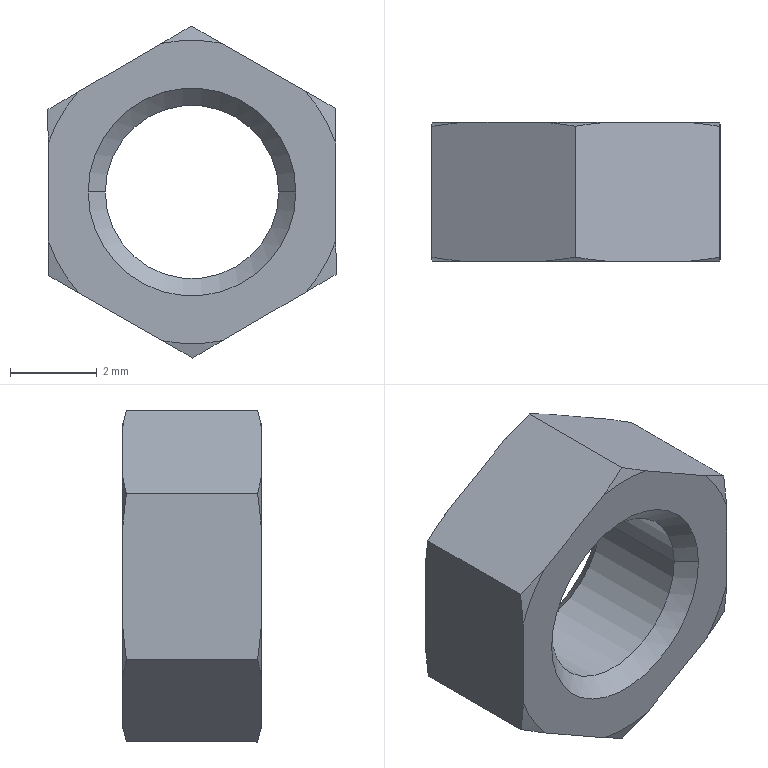Component | SolidWorks | GB_T6170-2000Type1HexNutGradeAAndBM4-1 | 1 solid | 26 faces | box 6.65 x 3.2 x 7.66 mm | volume 80 mm3 | cone 16 | plane 8 | cylinder 2 | commonest cylinder face diameters 4 x2
STEP:
#1=COLOUR_RGB('',0.7922,0.8196,0.9333);
#2=FILL_AREA_STYLE_COLOUR('',#1);
#3=FILL_AREA_STYLE('',(#2));
#4=SURFACE_STYLE_FILL_AREA(#3);
#5=SURFACE_SIDE_STYLE('',(#4));
#6=SURFACE_STYLE_USAGE(.BOTH.,#5);
#7=PRESENTATION_STYLE_ASSIGNMENT((#6));
#8=CARTESIAN_POINT('',(-5.651,2.991,-5.768));
#9=VERTEX_POINT('',#8);
#10=CARTESIAN_POINT('',(-5.493,2.991,-5.768));
#11=VERTEX_POINT('',#10);
#12=CARTESIAN_POINT('',(-5.572,2.991,-5.768));
#13=DIRECTION('',(0.,1.,0.));
#14=DIRECTION('',(-1.,0.,0.));
#15=AXIS2_PLACEMENT_3D('',#12,#13,#14);
#16=CIRCLE('',#15,0.07874);
#17=EDGE_CURVE('',#9,#11,#16,.T.);
#18=ORIENTED_EDGE('',*,*,#17,.F.);
#19=CARTESIAN_POINT('',(-5.667,3.007,-5.768));
#20=VERTEX_POINT('',#19);
#21=CARTESIAN_POINT('',(-5.651,2.991,-5.768));
#22=DIRECTION('',(-0.7071,0.7071,-0.));
#23=VECTOR('',#22,39.37);
#24=LINE('',#21,#23);
#25=EDGE_CURVE('',#9,#20,#24,.T.);
#26=ORIENTED_EDGE('',*,*,#25,.T.);
#27=CARTESIAN_POINT('',(-5.478,3.007,-5.768));
#28=VERTEX_POINT('',#27);
#29=CARTESIAN_POINT('',(-5.572,3.007,-5.768));
#30=DIRECTION('',(0.,-1.,0.));
#31=DIRECTION('',(-1.,0.,0.));
#32=AXIS2_PLACEMENT_3D('',#29,#30,#31);
#33=CIRCLE('',#32,0.0943);
#34=EDGE_CURVE('',#28,#20,#33,.T.);
#35=ORIENTED_EDGE('',*,*,#34,.F.);
#36=CARTESIAN_POINT('',(-5.493,2.991,-5.768));
#37=DIRECTION('',(0.7071,0.7071,0.));
#38=VECTOR('',#37,39.37);
#39=LINE('',#36,#38);
#40=EDGE_CURVE('',#11,#28,#39,.T.);
#41=ORIENTED_EDGE('',*,*,#40,.F.);
#42=EDGE_LOOP('',(#18,#26,#35,#41));
#43=FACE_OUTER_BOUND('',#42,.T.);
#44=CARTESIAN_POINT('',(-5.572,2.991,-5.768));
#45=DIRECTION('',(0.,1.,0.));
#46=DIRECTION('',(1.,0.,0.));
#47=AXIS2_PLACEMENT_3D('',#44,#45,#46);
#48=CONICAL_SURFACE('',#47,0.07874,0.7854);
#49=ADVANCED_FACE('',(#43),#48,.F.);
#50=CARTESIAN_POINT('',(-5.493,2.896,-5.768));
#51=VERTEX_POINT('',#50);
#52=CARTESIAN_POINT('',(-5.651,2.896,-5.768));
#53=VERTEX_POINT('',#52);
#54=CARTESIAN_POINT('',(-5.572,2.896,-5.768));
#55=DIRECTION('',(0.,-1.,0.));
#56=DIRECTION('',(-1.,0.,0.));
#57=AXIS2_PLACEMENT_3D('',#54,#55,#56);
#58=CIRCLE('',#57,0.07874);
#59=EDGE_CURVE('',#51,#53,#58,.T.);
#60=ORIENTED_EDGE('',*,*,#59,.F.);
#61=CARTESIAN_POINT('',(-5.478,2.881,-5.768));
#62=VERTEX_POINT('',#61);
#63=CARTESIAN_POINT('',(-5.478,2.881,-5.768));
#64=DIRECTION('',(0.7071,-0.7071,-0.));
#65=VECTOR('',#64,39.37);
#66=LINE('',#63,#65);
#67=EDGE_CURVE('',#51,#62,#66,.T.);
#68=ORIENTED_EDGE('',*,*,#67,.T.);
#69=CARTESIAN_POINT('',(-5.667,2.881,-5.768));
#70=VERTEX_POINT('',#69);
#71=CARTESIAN_POINT('',(-5.572,2.881,-5.768));
#72=DIRECTION('',(0.,1.,0.));
#73=DIRECTION('',(-1.,0.,0.));
#74=AXIS2_PLACEMENT_3D('',#71,#72,#73);
#75=CIRCLE('',#74,0.0943);
#76=EDGE_CURVE('',#70,#62,#75,.T.);
#77=ORIENTED_EDGE('',*,*,#76,.F.);
#78=CARTESIAN_POINT('',(-5.667,2.881,-5.768));
#79=DIRECTION('',(-0.7071,-0.7071,0.));
#80=VECTOR('',#79,39.37);
#81=LINE('',#78,#80);
#82=EDGE_CURVE('',#53,#70,#81,.T.);
#83=ORIENTED_EDGE('',*,*,#82,.F.);
#84=EDGE_LOOP('',(#60,#68,#77,#83));
#85=FACE_OUTER_BOUND('',#84,.T.);
#86=CARTESIAN_POINT('',(-5.572,2.881,-5.768));
#87=DIRECTION('',(0.,-1.,0.));
#88=DIRECTION('',(-1.,0.,0.));
#89=AXIS2_PLACEMENT_3D('',#86,#87,#88);
#90=CONICAL_SURFACE('',#89,0.0943,0.7854);
#91=ADVANCED_FACE('',(#85),#90,.F.);
#92=ORIENTED_EDGE('',*,*,#17,.T.);
#93=CARTESIAN_POINT('',(-5.493,3.007,-5.768));
#94=DIRECTION('',(0.,-1.,0.));
#95=VECTOR('',#94,39.37);
#96=LINE('',#93,#95);
#97=EDGE_CURVE('',#11,#51,#96,.T.);
#98=ORIENTED_EDGE('',*,*,#97,.T.);
#99=ORIENTED_EDGE('',*,*,#59,.T.);
#100=CARTESIAN_POINT('',(-5.651,3.007,-5.768));
#101=DIRECTION('',(0.,-1.,0.));
#102=VECTOR('',#101,39.37);
#103=LINE('',#100,#102);
#104=EDGE_CURVE('',#9,#53,#103,.T.);
#105=ORIENTED_EDGE('',*,*,#104,.F.);
#106=EDGE_LOOP('',(#92,#98,#99,#105));
#107=FACE_OUTER_BOUND('',#106,.T.);
#108=CARTESIAN_POINT('',(-5.572,3.007,-5.768));
#109=DIRECTION('',(0.,-1.,0.));
#110=DIRECTION('',(-1.,0.,0.));
#111=AXIS2_PLACEMENT_3D('',#108,#109,#110);
#112=CYLINDRICAL_SURFACE('',#111,0.07874);
#113=ADVANCED_FACE('',(#107),#112,.F.);
#114=CARTESIAN_POINT('',(-5.441,3.003,-5.843));
#115=VERTEX_POINT('',#114);
#116=CARTESIAN_POINT('',(-5.468,3.007,-5.859));
#117=VERTEX_POINT('',#116);
#118=CARTESIAN_POINT('',(-5.441,3.003,-5.843));
#119=CARTESIAN_POINT('',(-5.45,3.004,-5.848));
#120=CARTESIAN_POINT('',(-5.459,3.006,-5.853));
#121=CARTESIAN_POINT('',(-5.468,3.007,-5.859));
#122=B_SPLINE_CURVE_WITH_KNOTS('',3,(#118,#119,#120,#121),.UNSPECIFIED.,.F.,.F.,(4,4),(0.00352,0.004323),.UNSPECIFIED.);
#123=EDGE_CURVE('',#115,#117,#122,.T.);
#124=ORIENTED_EDGE('',*,*,#123,.F.);
#125=CARTESIAN_POINT('',(-5.441,2.884,-5.843));
#126=VERTEX_POINT('',#125);
#127=CARTESIAN_POINT('',(-5.441,3.007,-5.843));
#128=DIRECTION('',(0.,-1.,0.));
#129=VECTOR('',#128,39.37);
#130=LINE('',#127,#129);
#131=EDGE_CURVE('',#115,#126,#130,.T.);
#132=ORIENTED_EDGE('',*,*,#131,.T.);
#133=CARTESIAN_POINT('',(-5.468,2.881,-5.859));
#134=VERTEX_POINT('',#133);
#135=CARTESIAN_POINT('',(-5.468,2.881,-5.859));
#136=CARTESIAN_POINT('',(-5.459,2.881,-5.853));
#137=CARTESIAN_POINT('',(-5.45,2.883,-5.848));
#138=CARTESIAN_POINT('',(-5.441,2.884,-5.843));
#139=B_SPLINE_CURVE_WITH_KNOTS('',3,(#135,#136,#137,#138),.UNSPECIFIED.,.F.,.F.,(4,4),(0.006542,0.007331),.UNSPECIFIED.);
#140=EDGE_CURVE('',#134,#126,#139,.T.);
#141=ORIENTED_EDGE('',*,*,#140,.F.);
#142=CARTESIAN_POINT('',(-5.544,2.881,-5.903));
#143=VERTEX_POINT('',#142);
#144=CARTESIAN_POINT('',(-5.441,2.881,-5.843));
#145=DIRECTION('',(-0.8641,0.,-0.5034));
#146=VECTOR('',#145,39.37);
#147=LINE('',#144,#146);
#148=EDGE_CURVE('',#134,#143,#147,.T.);
#149=ORIENTED_EDGE('',*,*,#148,.T.);
#150=CARTESIAN_POINT('',(-5.572,2.884,-5.919));
#151=VERTEX_POINT('',#150);
#152=CARTESIAN_POINT('',(-5.572,2.884,-5.919));
#153=CARTESIAN_POINT('',(-5.563,2.883,-5.914));
#154=CARTESIAN_POINT('',(-5.554,2.881,-5.908));
#155=CARTESIAN_POINT('',(-5.544,2.881,-5.903));
#156=B_SPLINE_CURVE_WITH_KNOTS('',3,(#152,#153,#154,#155),.UNSPECIFIED.,.F.,.F.,(4,4),(0.00352,0.004323),.UNSPECIFIED.);
#157=EDGE_CURVE('',#151,#143,#156,.T.);
#158=ORIENTED_EDGE('',*,*,#157,.F.);
#159=CARTESIAN_POINT('',(-5.572,3.003,-5.919));
#160=VERTEX_POINT('',#159);
#161=CARTESIAN_POINT('',(-5.572,3.007,-5.919));
#162=DIRECTION('',(0.,-1.,0.));
#163=VECTOR('',#162,39.37);
#164=LINE('',#161,#163);
#165=EDGE_CURVE('',#160,#151,#164,.T.);
#166=ORIENTED_EDGE('',*,*,#165,.F.);
#167=CARTESIAN_POINT('',(-5.544,3.007,-5.903));
#168=VERTEX_POINT('',#167);
#169=CARTESIAN_POINT('',(-5.544,3.007,-5.903));
#170=CARTESIAN_POINT('',(-5.554,3.006,-5.908));
#171=CARTESIAN_POINT('',(-5.563,3.004,-5.914));
#172=CARTESIAN_POINT('',(-5.572,3.003,-5.919));
#173=B_SPLINE_CURVE_WITH_KNOTS('',3,(#169,#170,#171,#172),.UNSPECIFIED.,.F.,.F.,(4,4),(0.006542,0.007331),.UNSPECIFIED.);
#174=EDGE_CURVE('',#168,#160,#173,.T.);
#175=ORIENTED_EDGE('',*,*,#174,.F.);
#176=CARTESIAN_POINT('',(-5.441,3.007,-5.843));
#177=DIRECTION('',(-0.8641,0.,-0.5034));
#178=VECTOR('',#177,39.37);
#179=LINE('',#176,#178);
#180=EDGE_CURVE('',#117,#168,#179,.T.);
#181=ORIENTED_EDGE('',*,*,#180,.F.);
#182=EDGE_LOOP('',(#124,#132,#141,#149,#158,#166,#175,#181));
#183=FACE_OUTER_BOUND('',#182,.T.);
#184=CARTESIAN_POINT('',(-5.441,3.007,-5.843));
#185=DIRECTION('',(-0.5034,0.,0.8641));
#186=DIRECTION('',(0.8641,0.,0.5034));
#187=AXIS2_PLACEMENT_3D('',#184,#185,#186);
#188=PLANE('',#187);
#189=ADVANCED_FACE('',(#183),#188,.F.);
#190=CARTESIAN_POINT('',(-5.599,3.007,-5.903));
#191=VERTEX_POINT('',#190);
#192=CARTESIAN_POINT('',(-5.572,3.003,-5.919));
#193=CARTESIAN_POINT('',(-5.581,3.004,-5.914));
#194=CARTESIAN_POINT('',(-5.59,3.006,-5.908));
#195=CARTESIAN_POINT('',(-5.599,3.007,-5.903));
#196=B_SPLINE_CURVE_WITH_KNOTS('',3,(#192,#193,#194,#195),.UNSPECIFIED.,.F.,.F.,(4,4),(0.003504,0.004307),.UNSPECIFIED.);
#197=EDGE_CURVE('',#160,#191,#196,.T.);
#198=ORIENTED_EDGE('',*,*,#197,.F.);
#199=ORIENTED_EDGE('',*,*,#165,.T.);
#200=CARTESIAN_POINT('',(-5.599,2.881,-5.903));
#201=VERTEX_POINT('',#200);
#202=CARTESIAN_POINT('',(-5.599,2.881,-5.903));
#203=CARTESIAN_POINT('',(-5.59,2.881,-5.908));
#204=CARTESIAN_POINT('',(-5.581,2.883,-5.914));
#205=CARTESIAN_POINT('',(-5.572,2.884,-5.919));
#206=B_SPLINE_CURVE_WITH_KNOTS('',3,(#202,#203,#204,#205),.UNSPECIFIED.,.F.,.F.,(4,4),(0.006526,0.007315),.UNSPECIFIED.);
#207=EDGE_CURVE('',#201,#151,#206,.T.);
#208=ORIENTED_EDGE('',*,*,#207,.F.);
#209=CARTESIAN_POINT('',(-5.675,2.881,-5.859));
#210=VERTEX_POINT('',#209);
#211=CARTESIAN_POINT('',(-5.572,2.881,-5.919));
#212=DIRECTION('',(-0.868,0.,0.4966));
#213=VECTOR('',#212,39.37);
#214=LINE('',#211,#213);
#215=EDGE_CURVE('',#201,#210,#214,.T.);
#216=ORIENTED_EDGE('',*,*,#215,.T.);
#217=CARTESIAN_POINT('',(-5.703,2.884,-5.844));
#218=VERTEX_POINT('',#217);
#219=CARTESIAN_POINT('',(-5.703,2.884,-5.844));
#220=CARTESIAN_POINT('',(-5.693,2.883,-5.849));
#221=CARTESIAN_POINT('',(-5.684,2.881,-5.854));
#222=CARTESIAN_POINT('',(-5.675,2.881,-5.859));
#223=B_SPLINE_CURVE_WITH_KNOTS('',3,(#219,#220,#221,#222),.UNSPECIFIED.,.F.,.F.,(4,4),(0.003504,0.004307),.UNSPECIFIED.);
#224=EDGE_CURVE('',#218,#210,#223,.T.);
#225=ORIENTED_EDGE('',*,*,#224,.F.);
#226=CARTESIAN_POINT('',(-5.703,3.003,-5.844));
#227=VERTEX_POINT('',#226);
#228=CARTESIAN_POINT('',(-5.703,3.007,-5.844));
#229=DIRECTION('',(0.,-1.,0.));
#230=VECTOR('',#229,39.37);
#231=LINE('',#228,#230);
#232=EDGE_CURVE('',#227,#218,#231,.T.);
#233=ORIENTED_EDGE('',*,*,#232,.F.);
#234=CARTESIAN_POINT('',(-5.675,3.007,-5.859));
#235=VERTEX_POINT('',#234);
#236=CARTESIAN_POINT('',(-5.675,3.007,-5.859));
#237=CARTESIAN_POINT('',(-5.684,3.006,-5.854));
#238=CARTESIAN_POINT('',(-5.693,3.004,-5.849));
#239=CARTESIAN_POINT('',(-5.703,3.003,-5.844));
#240=B_SPLINE_CURVE_WITH_KNOTS('',3,(#236,#237,#238,#239),.UNSPECIFIED.,.F.,.F.,(4,4),(0.006526,0.007315),.UNSPECIFIED.);
#241=EDGE_CURVE('',#235,#227,#240,.T.);
#242=ORIENTED_EDGE('',*,*,#241,.F.);
#243=CARTESIAN_POINT('',(-5.572,3.007,-5.919));
#244=DIRECTION('',(-0.868,0.,0.4966));
#245=VECTOR('',#244,39.37);
#246=LINE('',#243,#245);
#247=EDGE_CURVE('',#191,#235,#246,.T.);
#248=ORIENTED_EDGE('',*,*,#247,.F.);
#249=EDGE_LOOP('',(#198,#199,#208,#216,#225,#233,#242,#248));
#250=FACE_OUTER_BOUND('',#249,.T.);
#251=CARTESIAN_POINT('',(-5.572,3.007,-5.919));
#252=DIRECTION('',(0.4966,0.,0.868));
#253=DIRECTION('',(0.868,0.,-0.4966));
#254=AXIS2_PLACEMENT_3D('',#251,#252,#253);
#255=PLANE('',#254);
#256=ADVANCED_FACE('',(#250),#255,.F.);
#257=CARTESIAN_POINT('',(-5.703,3.007,-5.812));
#258=VERTEX_POINT('',#257);
#259=CARTESIAN_POINT('',(-5.703,3.003,-5.844));
#260=CARTESIAN_POINT('',(-5.703,3.004,-5.833));
#261=CARTESIAN_POINT('',(-5.703,3.006,-5.823));
#262=CARTESIAN_POINT('',(-5.703,3.007,-5.812));
#263=B_SPLINE_CURVE_WITH_KNOTS('',3,(#259,#260,#261,#262),.UNSPECIFIED.,.F.,.F.,(4,4),(0.003038,0.00384),.UNSPECIFIED.);
#264=EDGE_CURVE('',#227,#258,#263,.T.);
#265=ORIENTED_EDGE('',*,*,#264,.F.);
#266=ORIENTED_EDGE('',*,*,#232,.T.);
#267=CARTESIAN_POINT('',(-5.703,2.881,-5.812));
#268=VERTEX_POINT('',#267);
#269=CARTESIAN_POINT('',(-5.703,2.881,-5.812));
#270=CARTESIAN_POINT('',(-5.703,2.881,-5.823));
#271=CARTESIAN_POINT('',(-5.703,2.883,-5.833));
#272=CARTESIAN_POINT('',(-5.703,2.884,-5.844));
#273=B_SPLINE_CURVE_WITH_KNOTS('',3,(#269,#270,#271,#272),.UNSPECIFIED.,.F.,.F.,(4,4),(0.006062,0.006851),.UNSPECIFIED.);
#274=EDGE_CURVE('',#268,#218,#273,.T.);
#275=ORIENTED_EDGE('',*,*,#274,.F.);
#276=CARTESIAN_POINT('',(-5.703,2.881,-5.725));
#277=VERTEX_POINT('',#276);
#278=CARTESIAN_POINT('',(-5.703,2.881,-5.844));
#279=DIRECTION('',(-0.003934,0.,1.));
#280=VECTOR('',#279,39.37);
#281=LINE('',#278,#280);
#282=EDGE_CURVE('',#268,#277,#281,.T.);
#283=ORIENTED_EDGE('',*,*,#282,.T.);
#284=CARTESIAN_POINT('',(-5.703,2.884,-5.693));
#285=VERTEX_POINT('',#284);
#286=CARTESIAN_POINT('',(-5.703,2.884,-5.693));
#287=CARTESIAN_POINT('',(-5.703,2.883,-5.704));
#288=CARTESIAN_POINT('',(-5.703,2.881,-5.714));
#289=CARTESIAN_POINT('',(-5.703,2.881,-5.725));
#290=B_SPLINE_CURVE_WITH_KNOTS('',3,(#286,#287,#288,#289),.UNSPECIFIED.,.F.,.F.,(4,4),(0.003038,0.00384),.UNSPECIFIED.);
#291=EDGE_CURVE('',#285,#277,#290,.T.);
#292=ORIENTED_EDGE('',*,*,#291,.F.);
#293=CARTESIAN_POINT('',(-5.703,3.003,-5.693));
#294=VERTEX_POINT('',#293);
#295=CARTESIAN_POINT('',(-5.703,3.007,-5.693));
#296=DIRECTION('',(0.,-1.,0.));
#297=VECTOR('',#296,39.37);
#298=LINE('',#295,#297);
#299=EDGE_CURVE('',#294,#285,#298,.T.);
#300=ORIENTED_EDGE('',*,*,#299,.F.);
#301=CARTESIAN_POINT('',(-5.703,3.007,-5.725));
#302=VERTEX_POINT('',#301);
#303=CARTESIAN_POINT('',(-5.703,3.007,-5.725));
#304=CARTESIAN_POINT('',(-5.703,3.006,-5.714));
#305=CARTESIAN_POINT('',(-5.703,3.004,-5.704));
#306=CARTESIAN_POINT('',(-5.703,3.003,-5.693));
#307=B_SPLINE_CURVE_WITH_KNOTS('',3,(#303,#304,#305,#306),.UNSPECIFIED.,.F.,.F.,(4,4),(0.006062,0.006851),.UNSPECIFIED.);
#308=EDGE_CURVE('',#302,#294,#307,.T.);
#309=ORIENTED_EDGE('',*,*,#308,.F.);
#310=CARTESIAN_POINT('',(-5.703,3.007,-5.844));
#311=DIRECTION('',(-0.003934,0.,1.));
#312=VECTOR('',#311,39.37);
#313=LINE('',#310,#312);
#314=EDGE_CURVE('',#258,#302,#313,.T.);
#315=ORIENTED_EDGE('',*,*,#314,.F.);
#316=EDGE_LOOP('',(#265,#266,#275,#283,#292,#300,#309,#315));
#317=FACE_OUTER_BOUND('',#316,.T.);
#318=CARTESIAN_POINT('',(-5.703,3.007,-5.844));
#319=DIRECTION('',(1.,0.,0.003934));
#320=DIRECTION('',(0.003934,0.,-1.));
#321=AXIS2_PLACEMENT_3D('',#318,#319,#320);
#322=PLANE('',#321);
#323=ADVANCED_FACE('',(#317),#322,.F.);
#324=CARTESIAN_POINT('',(-5.676,3.007,-5.677));
#325=VERTEX_POINT('',#324);
#326=CARTESIAN_POINT('',(-5.703,3.003,-5.693));
#327=CARTESIAN_POINT('',(-5.694,3.004,-5.688));
#328=CARTESIAN_POINT('',(-5.685,3.006,-5.683));
#329=CARTESIAN_POINT('',(-5.676,3.007,-5.677));
#330=B_SPLINE_CURVE_WITH_KNOTS('',3,(#326,#327,#328,#329),.UNSPECIFIED.,.F.,.F.,(4,4),(0.00352,0.004323),.UNSPECIFIED.);
#331=EDGE_CURVE('',#294,#325,#330,.T.);
#332=ORIENTED_EDGE('',*,*,#331,.F.);
#333=ORIENTED_EDGE('',*,*,#299,.T.);
#334=CARTESIAN_POINT('',(-5.676,2.881,-5.677));
#335=VERTEX_POINT('',#334);
#336=CARTESIAN_POINT('',(-5.676,2.881,-5.677));
#337=CARTESIAN_POINT('',(-5.685,2.881,-5.683));
#338=CARTESIAN_POINT('',(-5.694,2.883,-5.688));
#339=CARTESIAN_POINT('',(-5.703,2.884,-5.693));
#340=B_SPLINE_CURVE_WITH_KNOTS('',3,(#336,#337,#338,#339),.UNSPECIFIED.,.F.,.F.,(4,4),(0.006542,0.007331),.UNSPECIFIED.);
#341=EDGE_CURVE('',#335,#285,#340,.T.);
#342=ORIENTED_EDGE('',*,*,#341,.F.);
#343=CARTESIAN_POINT('',(-5.6,2.881,-5.633));
#344=VERTEX_POINT('',#343);
#345=CARTESIAN_POINT('',(-5.703,2.881,-5.693));
#346=DIRECTION('',(0.8641,0.,0.5034));
#347=VECTOR('',#346,39.37);
#348=LINE('',#345,#347);
#349=EDGE_CURVE('',#335,#344,#348,.T.);
#350=ORIENTED_EDGE('',*,*,#349,.T.);
#351=CARTESIAN_POINT('',(-5.573,2.884,-5.617));
#352=VERTEX_POINT('',#351);
#353=CARTESIAN_POINT('',(-5.573,2.884,-5.617));
#354=CARTESIAN_POINT('',(-5.582,2.883,-5.622));
#355=CARTESIAN_POINT('',(-5.591,2.881,-5.628));
#356=CARTESIAN_POINT('',(-5.6,2.881,-5.633));
#357=B_SPLINE_CURVE_WITH_KNOTS('',3,(#353,#354,#355,#356),.UNSPECIFIED.,.F.,.F.,(4,4),(0.00352,0.004323),.UNSPECIFIED.);
#358=EDGE_CURVE('',#352,#344,#357,.T.);
#359=ORIENTED_EDGE('',*,*,#358,.F.);
#360=CARTESIAN_POINT('',(-5.573,3.003,-5.617));
#361=VERTEX_POINT('',#360);
#362=CARTESIAN_POINT('',(-5.573,3.007,-5.617));
#363=DIRECTION('',(0.,-1.,0.));
#364=VECTOR('',#363,39.37);
#365=LINE('',#362,#364);
#366=EDGE_CURVE('',#361,#352,#365,.T.);
#367=ORIENTED_EDGE('',*,*,#366,.F.);
#368=CARTESIAN_POINT('',(-5.6,3.007,-5.633));
#369=VERTEX_POINT('',#368);
#370=CARTESIAN_POINT('',(-5.6,3.007,-5.633));
#371=CARTESIAN_POINT('',(-5.591,3.006,-5.628));
#372=CARTESIAN_POINT('',(-5.582,3.004,-5.622));
#373=CARTESIAN_POINT('',(-5.573,3.003,-5.617));
#374=B_SPLINE_CURVE_WITH_KNOTS('',3,(#370,#371,#372,#373),.UNSPECIFIED.,.F.,.F.,(4,4),(0.006542,0.007331),.UNSPECIFIED.);
#375=EDGE_CURVE('',#369,#361,#374,.T.);
#376=ORIENTED_EDGE('',*,*,#375,.F.);
#377=CARTESIAN_POINT('',(-5.703,3.007,-5.693));
#378=DIRECTION('',(0.8641,0.,0.5034));
#379=VECTOR('',#378,39.37);
#380=LINE('',#377,#379);
#381=EDGE_CURVE('',#325,#369,#380,.T.);
#382=ORIENTED_EDGE('',*,*,#381,.F.);
#383=EDGE_LOOP('',(#332,#333,#342,#350,#359,#367,#376,#382));
#384=FACE_OUTER_BOUND('',#383,.T.);
#385=CARTESIAN_POINT('',(-5.703,3.007,-5.693));
#386=DIRECTION('',(0.5034,0.,-0.8641));
#387=DIRECTION('',(-0.8641,0.,-0.5034));
#388=AXIS2_PLACEMENT_3D('',#385,#386,#387);
#389=PLANE('',#388);
#390=ADVANCED_FACE('',(#384),#389,.F.);
#391=CARTESIAN_POINT('',(-5.546,3.007,-5.633));
#392=VERTEX_POINT('',#391);
#393=CARTESIAN_POINT('',(-5.573,3.003,-5.617));
#394=CARTESIAN_POINT('',(-5.564,3.004,-5.622));
#395=CARTESIAN_POINT('',(-5.555,3.006,-5.628));
#396=CARTESIAN_POINT('',(-5.546,3.007,-5.633));
#397=B_SPLINE_CURVE_WITH_KNOTS('',3,(#393,#394,#395,#396),.UNSPECIFIED.,.F.,.F.,(4,4),(0.003504,0.004307),.UNSPECIFIED.);
#398=EDGE_CURVE('',#361,#392,#397,.T.);
#399=ORIENTED_EDGE('',*,*,#398,.F.);
#400=ORIENTED_EDGE('',*,*,#366,.T.);
#401=CARTESIAN_POINT('',(-5.546,2.881,-5.633));
#402=VERTEX_POINT('',#401);
#403=CARTESIAN_POINT('',(-5.546,2.881,-5.633));
#404=CARTESIAN_POINT('',(-5.555,2.881,-5.628));
#405=CARTESIAN_POINT('',(-5.564,2.883,-5.622));
#406=CARTESIAN_POINT('',(-5.573,2.884,-5.617));
#407=B_SPLINE_CURVE_WITH_KNOTS('',3,(#403,#404,#405,#406),.UNSPECIFIED.,.F.,.F.,(4,4),(0.006526,0.007315),.UNSPECIFIED.);
#408=EDGE_CURVE('',#402,#352,#407,.T.);
#409=ORIENTED_EDGE('',*,*,#408,.F.);
#410=CARTESIAN_POINT('',(-5.469,2.881,-5.676));
#411=VERTEX_POINT('',#410);
#412=CARTESIAN_POINT('',(-5.573,2.881,-5.617));
#413=DIRECTION('',(0.868,0.,-0.4966));
#414=VECTOR('',#413,39.37);
#415=LINE('',#412,#414);
#416=EDGE_CURVE('',#402,#411,#415,.T.);
#417=ORIENTED_EDGE('',*,*,#416,.T.);
#418=CARTESIAN_POINT('',(-5.442,2.884,-5.692));
#419=VERTEX_POINT('',#418);
#420=CARTESIAN_POINT('',(-5.442,2.884,-5.692));
#421=CARTESIAN_POINT('',(-5.451,2.883,-5.687));
#422=CARTESIAN_POINT('',(-5.46,2.881,-5.682));
#423=CARTESIAN_POINT('',(-5.469,2.881,-5.676));
#424=B_SPLINE_CURVE_WITH_KNOTS('',3,(#420,#421,#422,#423),.UNSPECIFIED.,.F.,.F.,(4,4),(0.003504,0.004307),.UNSPECIFIED.);
#425=EDGE_CURVE('',#419,#411,#424,.T.);
#426=ORIENTED_EDGE('',*,*,#425,.F.);
#427=CARTESIAN_POINT('',(-5.442,3.003,-5.692));
#428=VERTEX_POINT('',#427);
#429=CARTESIAN_POINT('',(-5.442,3.007,-5.692));
#430=DIRECTION('',(0.,-1.,0.));
#431=VECTOR('',#430,39.37);
#432=LINE('',#429,#431);
#433=EDGE_CURVE('',#428,#419,#432,.T.);
#434=ORIENTED_EDGE('',*,*,#433,.F.);
#435=CARTESIAN_POINT('',(-5.469,3.007,-5.676));
#436=VERTEX_POINT('',#435);
#437=CARTESIAN_POINT('',(-5.469,3.007,-5.676));
#438=CARTESIAN_POINT('',(-5.46,3.006,-5.682));
#439=CARTESIAN_POINT('',(-5.451,3.004,-5.687));
#440=CARTESIAN_POINT('',(-5.442,3.003,-5.692));
#441=B_SPLINE_CURVE_WITH_KNOTS('',3,(#437,#438,#439,#440),.UNSPECIFIED.,.F.,.F.,(4,4),(0.006526,0.007315),.UNSPECIFIED.);
#442=EDGE_CURVE('',#436,#428,#441,.T.);
#443=ORIENTED_EDGE('',*,*,#442,.F.);
#444=CARTESIAN_POINT('',(-5.573,3.007,-5.617));
#445=DIRECTION('',(0.868,0.,-0.4966));
#446=VECTOR('',#445,39.37);
#447=LINE('',#444,#446);
#448=EDGE_CURVE('',#392,#436,#447,.T.);
#449=ORIENTED_EDGE('',*,*,#448,.F.);
#450=EDGE_LOOP('',(#399,#400,#409,#417,#426,#434,#443,#449));
#451=FACE_OUTER_BOUND('',#450,.T.);
#452=CARTESIAN_POINT('',(-5.573,3.007,-5.617));
#453=DIRECTION('',(-0.4966,0.,-0.868));
#454=DIRECTION('',(-0.868,0.,0.4966));
#455=AXIS2_PLACEMENT_3D('',#452,#453,#454);
#456=PLANE('',#455);
#457=ADVANCED_FACE('',(#451),#456,.F.);
#458=CARTESIAN_POINT('',(-5.442,3.007,-5.723));
#459=VERTEX_POINT('',#458);
#460=CARTESIAN_POINT('',(-5.442,3.003,-5.692));
#461=CARTESIAN_POINT('',(-5.442,3.004,-5.703));
#462=CARTESIAN_POINT('',(-5.442,3.006,-5.713));
#463=CARTESIAN_POINT('',(-5.442,3.007,-5.723));
#464=B_SPLINE_CURVE_WITH_KNOTS('',3,(#460,#461,#462,#463),.UNSPECIFIED.,.F.,.F.,(4,4),(0.003038,0.00384),.UNSPECIFIED.);
#465=EDGE_CURVE('',#428,#459,#464,.T.);
#466=ORIENTED_EDGE('',*,*,#465,.F.);
#467=ORIENTED_EDGE('',*,*,#433,.T.);
#468=CARTESIAN_POINT('',(-5.442,2.881,-5.723));
#469=VERTEX_POINT('',#468);
#470=CARTESIAN_POINT('',(-5.442,2.881,-5.723));
#471=CARTESIAN_POINT('',(-5.442,2.881,-5.713));
#472=CARTESIAN_POINT('',(-5.442,2.883,-5.703));
#473=CARTESIAN_POINT('',(-5.442,2.884,-5.692));
#474=B_SPLINE_CURVE_WITH_KNOTS('',3,(#470,#471,#472,#473),.UNSPECIFIED.,.F.,.F.,(4,4),(0.006062,0.006851),.UNSPECIFIED.);
#475=EDGE_CURVE('',#469,#419,#474,.T.);
#476=ORIENTED_EDGE('',*,*,#475,.F.);
#477=CARTESIAN_POINT('',(-5.441,2.881,-5.811));
#478=VERTEX_POINT('',#477);
#479=CARTESIAN_POINT('',(-5.442,2.881,-5.692));
#480=DIRECTION('',(0.003934,0.,-1.));
#481=VECTOR('',#480,39.37);
#482=LINE('',#479,#481);
#483=EDGE_CURVE('',#469,#478,#482,.T.);
#484=ORIENTED_EDGE('',*,*,#483,.T.);
#485=CARTESIAN_POINT('',(-5.441,2.884,-5.843));
#486=CARTESIAN_POINT('',(-5.441,2.883,-5.832));
#487=CARTESIAN_POINT('',(-5.441,2.881,-5.822));
#488=CARTESIAN_POINT('',(-5.441,2.881,-5.811));
#489=B_SPLINE_CURVE_WITH_KNOTS('',3,(#485,#486,#487,#488),.UNSPECIFIED.,.F.,.F.,(4,4),(0.003038,0.00384),.UNSPECIFIED.);
#490=EDGE_CURVE('',#126,#478,#489,.T.);
#491=ORIENTED_EDGE('',*,*,#490,.F.);
#492=ORIENTED_EDGE('',*,*,#131,.F.);
#493=CARTESIAN_POINT('',(-5.441,3.007,-5.811));
#494=VERTEX_POINT('',#493);
#495=CARTESIAN_POINT('',(-5.441,3.007,-5.811));
#496=CARTESIAN_POINT('',(-5.441,3.006,-5.822));
#497=CARTESIAN_POINT('',(-5.441,3.004,-5.832));
#498=CARTESIAN_POINT('',(-5.441,3.003,-5.843));
#499=B_SPLINE_CURVE_WITH_KNOTS('',3,(#495,#496,#497,#498),.UNSPECIFIED.,.F.,.F.,(4,4),(0.006062,0.006851),.UNSPECIFIED.);
#500=EDGE_CURVE('',#494,#115,#499,.T.);
#501=ORIENTED_EDGE('',*,*,#500,.F.);
#502=CARTESIAN_POINT('',(-5.442,3.007,-5.692));
#503=DIRECTION('',(0.003934,0.,-1.));
#504=VECTOR('',#503,39.37);
#505=LINE('',#502,#504);
#506=EDGE_CURVE('',#459,#494,#505,.T.);
#507=ORIENTED_EDGE('',*,*,#506,.F.);
#508=EDGE_LOOP('',(#466,#467,#476,#484,#491,#492,#501,#507));
#509=FACE_OUTER_BOUND('',#508,.T.);
#510=CARTESIAN_POINT('',(-5.442,3.007,-5.692));
#511=DIRECTION('',(-1.,0.,-0.003934));
#512=DIRECTION('',(-0.003934,0.,1.));
#513=AXIS2_PLACEMENT_3D('',#510,#511,#512);
#514=PLANE('',#513);
#515=ADVANCED_FACE('',(#509),#514,.F.);
#516=ORIENTED_EDGE('',*,*,#34,.T.);
#517=CARTESIAN_POINT('',(-5.572,3.007,-5.768));
#518=DIRECTION('',(0.,-1.,0.));
#519=DIRECTION('',(-1.,0.,0.));
#520=AXIS2_PLACEMENT_3D('',#517,#518,#519);
#521=CIRCLE('',#520,0.0943);
#522=EDGE_CURVE('',#20,#28,#521,.T.);
#523=ORIENTED_EDGE('',*,*,#522,.T.);
#524=EDGE_LOOP('',(#516,#523));
#525=FACE_BOUND('',#524,.T.);
#526=CARTESIAN_POINT('',(-5.572,3.007,-5.768));
#527=DIRECTION('',(0.,-1.,0.));
#528=DIRECTION('',(-1.,0.,0.));
#529=AXIS2_PLACEMENT_3D('',#526,#527,#528);
#530=CIRCLE('',#529,0.1378);
#531=EDGE_CURVE('',#258,#235,#530,.T.);
#532=ORIENTED_EDGE('',*,*,#531,.F.);
#533=ORIENTED_EDGE('',*,*,#314,.T.);
#534=CARTESIAN_POINT('',(-5.572,3.007,-5.768));
#535=DIRECTION('',(0.,-1.,0.));
#536=DIRECTION('',(-1.,0.,0.));
#537=AXIS2_PLACEMENT_3D('',#534,#535,#536);
#538=CIRCLE('',#537,0.1378);
#539=EDGE_CURVE('',#325,#302,#538,.T.);
#540=ORIENTED_EDGE('',*,*,#539,.F.);
#541=ORIENTED_EDGE('',*,*,#381,.T.);
#542=CARTESIAN_POINT('',(-5.572,3.007,-5.768));
#543=DIRECTION('',(0.,-1.,0.));
#544=DIRECTION('',(-1.,0.,0.));
#545=AXIS2_PLACEMENT_3D('',#542,#543,#544);
#546=CIRCLE('',#545,0.1378);
#547=EDGE_CURVE('',#392,#369,#546,.T.);
#548=ORIENTED_EDGE('',*,*,#547,.F.);
#549=ORIENTED_EDGE('',*,*,#448,.T.);
#550=CARTESIAN_POINT('',(-5.572,3.007,-5.768));
#551=DIRECTION('',(0.,-1.,0.));
#552=DIRECTION('',(-1.,0.,0.));
#553=AXIS2_PLACEMENT_3D('',#550,#551,#552);
#554=CIRCLE('',#553,0.1378);
#555=EDGE_CURVE('',#459,#436,#554,.T.);
#556=ORIENTED_EDGE('',*,*,#555,.F.);
#557=ORIENTED_EDGE('',*,*,#506,.T.);
#558=CARTESIAN_POINT('',(-5.572,3.007,-5.768));
#559=DIRECTION('',(0.,1.,0.));
#560=DIRECTION('',(1.,0.,0.));
#561=AXIS2_PLACEMENT_3D('',#558,#559,#560);
#562=CIRCLE('',#561,0.1378);
#563=EDGE_CURVE('',#494,#117,#562,.T.);
#564=ORIENTED_EDGE('',*,*,#563,.T.);
#565=ORIENTED_EDGE('',*,*,#180,.T.);
#566=CARTESIAN_POINT('',(-5.572,3.007,-5.768));
#567=DIRECTION('',(0.,-1.,0.));
#568=DIRECTION('',(-1.,0.,0.));
#569=AXIS2_PLACEMENT_3D('',#566,#567,#568);
#570=CIRCLE('',#569,0.1378);
#571=EDGE_CURVE('',#191,#168,#570,.T.);
#572=ORIENTED_EDGE('',*,*,#571,.F.);
#573=ORIENTED_EDGE('',*,*,#247,.T.);
#574=EDGE_LOOP('',(#532,#533,#540,#541,#548,#549,#556,#557,#564,#565,#572,#573));
#575=FACE_OUTER_BOUND('',#574,.T.);
#576=CARTESIAN_POINT('',(-5.311,3.007,-5.767));
#577=DIRECTION('',(0.,-1.,0.));
#578=DIRECTION('',(-1.,0.,0.));
#579=AXIS2_PLACEMENT_3D('',#576,#577,#578);
#580=PLANE('',#579);
#581=ADVANCED_FACE('',(#525,#575),#580,.F.);
#582=ORIENTED_EDGE('',*,*,#76,.T.);
#583=CARTESIAN_POINT('',(-5.572,2.881,-5.768));
#584=DIRECTION('',(0.,1.,0.));
#585=DIRECTION('',(-1.,0.,0.));
#586=AXIS2_PLACEMENT_3D('',#583,#584,#585);
#587=CIRCLE('',#586,0.0943);
#588=EDGE_CURVE('',#62,#70,#587,.T.);
#589=ORIENTED_EDGE('',*,*,#588,.T.);
#590=EDGE_LOOP('',(#582,#589));
#591=FACE_BOUND('',#590,.T.);
#592=ORIENTED_EDGE('',*,*,#282,.F.);
#593=CARTESIAN_POINT('',(-5.572,2.881,-5.768));
#594=DIRECTION('',(0.,-1.,0.));
#595=DIRECTION('',(-1.,0.,0.));
#596=AXIS2_PLACEMENT_3D('',#593,#594,#595);
#597=CIRCLE('',#596,0.1378);
#598=EDGE_CURVE('',#268,#210,#597,.T.);
#599=ORIENTED_EDGE('',*,*,#598,.T.);
#600=ORIENTED_EDGE('',*,*,#215,.F.);
#601=CARTESIAN_POINT('',(-5.572,2.881,-5.768));
#602=DIRECTION('',(0.,-1.,0.));
#603=DIRECTION('',(-1.,0.,0.));
#604=AXIS2_PLACEMENT_3D('',#601,#602,#603);
#605=CIRCLE('',#604,0.1378);
#606=EDGE_CURVE('',#201,#143,#605,.T.);
#607=ORIENTED_EDGE('',*,*,#606,.T.);
#608=ORIENTED_EDGE('',*,*,#148,.F.);
#609=CARTESIAN_POINT('',(-5.572,2.881,-5.768));
#610=DIRECTION('',(0.,-1.,0.));
#611=DIRECTION('',(-1.,0.,0.));
#612=AXIS2_PLACEMENT_3D('',#609,#610,#611);
#613=CIRCLE('',#612,0.1378);
#614=EDGE_CURVE('',#134,#478,#613,.T.);
#615=ORIENTED_EDGE('',*,*,#614,.T.);
#616=ORIENTED_EDGE('',*,*,#483,.F.);
#617=CARTESIAN_POINT('',(-5.572,2.881,-5.768));
#618=DIRECTION('',(0.,-1.,0.));
#619=DIRECTION('',(-1.,0.,0.));
#620=AXIS2_PLACEMENT_3D('',#617,#618,#619);
#621=CIRCLE('',#620,0.1378);
#622=EDGE_CURVE('',#469,#411,#621,.T.);
#623=ORIENTED_EDGE('',*,*,#622,.T.);
#624=ORIENTED_EDGE('',*,*,#416,.F.);
#625=CARTESIAN_POINT('',(-5.572,2.881,-5.768));
#626=DIRECTION('',(0.,-1.,0.));
#627=DIRECTION('',(-1.,0.,0.));
#628=AXIS2_PLACEMENT_3D('',#625,#626,#627);
#629=CIRCLE('',#628,0.1378);
#630=EDGE_CURVE('',#402,#344,#629,.T.);
#631=ORIENTED_EDGE('',*,*,#630,.T.);
#632=ORIENTED_EDGE('',*,*,#349,.F.);
#633=CARTESIAN_POINT('',(-5.572,2.881,-5.768));
#634=DIRECTION('',(0.,-1.,0.));
#635=DIRECTION('',(-1.,0.,0.));
#636=AXIS2_PLACEMENT_3D('',#633,#634,#635);
#637=CIRCLE('',#636,0.1378);
#638=EDGE_CURVE('',#335,#277,#637,.T.);
#639=ORIENTED_EDGE('',*,*,#638,.T.);
#640=EDGE_LOOP('',(#592,#599,#600,#607,#608,#615,#616,#623,#624,#631,#632,#639));
#641=FACE_OUTER_BOUND('',#640,.T.);
#642=CARTESIAN_POINT('',(-5.311,2.881,-5.767));
#643=DIRECTION('',(0.,-1.,0.));
#644=DIRECTION('',(-1.,0.,0.));
#645=AXIS2_PLACEMENT_3D('',#642,#643,#644);
#646=PLANE('',#645);
#647=ADVANCED_FACE('',(#591,#641),#646,.T.);
#648=ORIENTED_EDGE('',*,*,#97,.F.);
#649=CARTESIAN_POINT('',(-5.572,2.991,-5.768));
#650=DIRECTION('',(0.,1.,0.));
#651=DIRECTION('',(-1.,0.,0.));
#652=AXIS2_PLACEMENT_3D('',#649,#650,#651);
#653=CIRCLE('',#652,0.07874);
#654=EDGE_CURVE('',#11,#9,#653,.T.);
#655=ORIENTED_EDGE('',*,*,#654,.T.);
#656=ORIENTED_EDGE('',*,*,#104,.T.);
#657=CARTESIAN_POINT('',(-5.572,2.896,-5.768));
#658=DIRECTION('',(0.,-1.,0.));
#659=DIRECTION('',(-1.,0.,0.));
#660=AXIS2_PLACEMENT_3D('',#657,#658,#659);
#661=CIRCLE('',#660,0.07874);
#662=EDGE_CURVE('',#53,#51,#661,.T.);
#663=ORIENTED_EDGE('',*,*,#662,.T.);
#664=EDGE_LOOP('',(#648,#655,#656,#663));
#665=FACE_OUTER_BOUND('',#664,.T.);
#666=CARTESIAN_POINT('',(-5.572,3.007,-5.768));
#667=DIRECTION('',(0.,-1.,0.));
#668=DIRECTION('',(-1.,0.,0.));
#669=AXIS2_PLACEMENT_3D('',#666,#667,#668);
#670=CYLINDRICAL_SURFACE('',#669,0.07874);
#671=ADVANCED_FACE('',(#665),#670,.F.);
#672=ORIENTED_EDGE('',*,*,#425,.T.);
#673=ORIENTED_EDGE('',*,*,#622,.F.);
#674=ORIENTED_EDGE('',*,*,#475,.T.);
#675=EDGE_LOOP('',(#672,#673,#674));
#676=FACE_OUTER_BOUND('',#675,.T.);
#677=CARTESIAN_POINT('',(-5.572,2.881,-5.768));
#678=DIRECTION('',(0.,1.,0.));
#679=DIRECTION('',(-1.,0.,0.));
#680=AXIS2_PLACEMENT_3D('',#677,#678,#679);
#681=CONICAL_SURFACE('',#680,0.1378,1.309);
#682=ADVANCED_FACE('',(#676),#681,.T.);
#683=ORIENTED_EDGE('',*,*,#140,.T.);
#684=ORIENTED_EDGE('',*,*,#490,.T.);
#685=ORIENTED_EDGE('',*,*,#614,.F.);
#686=EDGE_LOOP('',(#683,#684,#685));
#687=FACE_OUTER_BOUND('',#686,.T.);
#688=CARTESIAN_POINT('',(-5.572,2.881,-5.768));
#689=DIRECTION('',(0.,1.,0.));
#690=DIRECTION('',(-1.,0.,0.));
#691=AXIS2_PLACEMENT_3D('',#688,#689,#690);
#692=CONICAL_SURFACE('',#691,0.1378,1.309);
#693=ADVANCED_FACE('',(#687),#692,.T.);
#694=ORIENTED_EDGE('',*,*,#358,.T.);
#695=ORIENTED_EDGE('',*,*,#630,.F.);
#696=ORIENTED_EDGE('',*,*,#408,.T.);
#697=EDGE_LOOP('',(#694,#695,#696));
#698=FACE_OUTER_BOUND('',#697,.T.);
#699=CARTESIAN_POINT('',(-5.572,2.881,-5.768));
#700=DIRECTION('',(0.,1.,0.));
#701=DIRECTION('',(-1.,0.,0.));
#702=AXIS2_PLACEMENT_3D('',#699,#700,#701);
#703=CONICAL_SURFACE('',#702,0.1378,1.309);
#704=ADVANCED_FACE('',(#698),#703,.T.);
#705=ORIENTED_EDGE('',*,*,#291,.T.);
#706=ORIENTED_EDGE('',*,*,#638,.F.);
#707=ORIENTED_EDGE('',*,*,#341,.T.);
#708=EDGE_LOOP('',(#705,#706,#707));
#709=FACE_OUTER_BOUND('',#708,.T.);
#710=CARTESIAN_POINT('',(-5.572,2.881,-5.768));
#711=DIRECTION('',(0.,1.,0.));
#712=DIRECTION('',(-1.,0.,0.));
#713=AXIS2_PLACEMENT_3D('',#710,#711,#712);
#714=CONICAL_SURFACE('',#713,0.1378,1.309);
#715=ADVANCED_FACE('',(#709),#714,.T.);
#716=ORIENTED_EDGE('',*,*,#224,.T.);
#717=ORIENTED_EDGE('',*,*,#598,.F.);
#718=ORIENTED_EDGE('',*,*,#274,.T.);
#719=EDGE_LOOP('',(#716,#717,#718));
#720=FACE_OUTER_BOUND('',#719,.T.);
#721=CARTESIAN_POINT('',(-5.572,2.881,-5.768));
#722=DIRECTION('',(0.,1.,0.));
#723=DIRECTION('',(-1.,0.,0.));
#724=AXIS2_PLACEMENT_3D('',#721,#722,#723);
#725=CONICAL_SURFACE('',#724,0.1378,1.309);
#726=ADVANCED_FACE('',(#720),#725,.T.);
#727=ORIENTED_EDGE('',*,*,#157,.T.);
#728=ORIENTED_EDGE('',*,*,#606,.F.);
#729=ORIENTED_EDGE('',*,*,#207,.T.);
#730=EDGE_LOOP('',(#727,#728,#729));
#731=FACE_OUTER_BOUND('',#730,.T.);
#732=CARTESIAN_POINT('',(-5.572,2.881,-5.768));
#733=DIRECTION('',(0.,1.,0.));
#734=DIRECTION('',(-1.,0.,0.));
#735=AXIS2_PLACEMENT_3D('',#732,#733,#734);
#736=CONICAL_SURFACE('',#735,0.1378,1.309);
#737=ADVANCED_FACE('',(#731),#736,.T.);
#738=ORIENTED_EDGE('',*,*,#308,.T.);
#739=ORIENTED_EDGE('',*,*,#331,.T.);
#740=ORIENTED_EDGE('',*,*,#539,.T.);
#741=EDGE_LOOP('',(#738,#739,#740));
#742=FACE_OUTER_BOUND('',#741,.T.);
#743=CARTESIAN_POINT('',(-5.572,3.007,-5.768));
#744=DIRECTION('',(0.,-1.,0.));
#745=DIRECTION('',(1.,0.,0.));
#746=AXIS2_PLACEMENT_3D('',#743,#744,#745);
#747=CONICAL_SURFACE('',#746,0.1378,1.309);
#748=ADVANCED_FACE('',(#742),#747,.T.);
#749=ORIENTED_EDGE('',*,*,#375,.T.);
#750=ORIENTED_EDGE('',*,*,#398,.T.);
#751=ORIENTED_EDGE('',*,*,#547,.T.);
#752=EDGE_LOOP('',(#749,#750,#751));
#753=FACE_OUTER_BOUND('',#752,.T.);
#754=CARTESIAN_POINT('',(-5.572,3.007,-5.768));
#755=DIRECTION('',(0.,-1.,0.));
#756=DIRECTION('',(1.,0.,0.));
#757=AXIS2_PLACEMENT_3D('',#754,#755,#756);
#758=CONICAL_SURFACE('',#757,0.1378,1.309);
#759=ADVANCED_FACE('',(#753),#758,.T.);
#760=ORIENTED_EDGE('',*,*,#442,.T.);
#761=ORIENTED_EDGE('',*,*,#465,.T.);
#762=ORIENTED_EDGE('',*,*,#555,.T.);
#763=EDGE_LOOP('',(#760,#761,#762));
#764=FACE_OUTER_BOUND('',#763,.T.);
#765=CARTESIAN_POINT('',(-5.572,3.007,-5.768));
#766=DIRECTION('',(0.,-1.,0.));
#767=DIRECTION('',(1.,0.,0.));
#768=AXIS2_PLACEMENT_3D('',#765,#766,#767);
#769=CONICAL_SURFACE('',#768,0.1378,1.309);
#770=ADVANCED_FACE('',(#764),#769,.T.);
#771=ORIENTED_EDGE('',*,*,#123,.T.);
#772=ORIENTED_EDGE('',*,*,#563,.F.);
#773=ORIENTED_EDGE('',*,*,#500,.T.);
#774=EDGE_LOOP('',(#771,#772,#773));
#775=FACE_OUTER_BOUND('',#774,.T.);
#776=CARTESIAN_POINT('',(-5.572,3.007,-5.768));
#777=DIRECTION('',(0.,-1.,0.));
#778=DIRECTION('',(1.,0.,0.));
#779=AXIS2_PLACEMENT_3D('',#776,#777,#778);
#780=CONICAL_SURFACE('',#779,0.1378,1.309);
#781=ADVANCED_FACE('',(#775),#780,.T.);
#782=ORIENTED_EDGE('',*,*,#174,.T.);
#783=ORIENTED_EDGE('',*,*,#197,.T.);
#784=ORIENTED_EDGE('',*,*,#571,.T.);
#785=EDGE_LOOP('',(#782,#783,#784));
#786=FACE_OUTER_BOUND('',#785,.T.);
#787=CARTESIAN_POINT('',(-5.572,3.007,-5.768));
#788=DIRECTION('',(0.,-1.,0.));
#789=DIRECTION('',(1.,0.,0.));
#790=AXIS2_PLACEMENT_3D('',#787,#788,#789);
#791=CONICAL_SURFACE('',#790,0.1378,1.309);
#792=ADVANCED_FACE('',(#786),#791,.T.);
#793=ORIENTED_EDGE('',*,*,#241,.T.);
#794=ORIENTED_EDGE('',*,*,#264,.T.);
#795=ORIENTED_EDGE('',*,*,#531,.T.);
#796=EDGE_LOOP('',(#793,#794,#795));
#797=FACE_OUTER_BOUND('',#796,.T.);
#798=CARTESIAN_POINT('',(-5.572,3.007,-5.768));
#799=DIRECTION('',(0.,-1.,0.));
#800=DIRECTION('',(1.,0.,0.));
#801=AXIS2_PLACEMENT_3D('',#798,#799,#800);
#802=CONICAL_SURFACE('',#801,0.1378,1.309);
#803=ADVANCED_FACE('',(#797),#802,.T.);
#804=ORIENTED_EDGE('',*,*,#67,.F.);
#805=ORIENTED_EDGE('',*,*,#662,.F.);
#806=ORIENTED_EDGE('',*,*,#82,.T.);
#807=ORIENTED_EDGE('',*,*,#588,.F.);
#808=EDGE_LOOP('',(#804,#805,#806,#807));
#809=FACE_OUTER_BOUND('',#808,.T.);
#810=CARTESIAN_POINT('',(-5.572,2.881,-5.768));
#811=DIRECTION('',(0.,-1.,0.));
#812=DIRECTION('',(-1.,0.,0.));
#813=AXIS2_PLACEMENT_3D('',#810,#811,#812);
#814=CONICAL_SURFACE('',#813,0.0943,0.7854);
#815=ADVANCED_FACE('',(#809),#814,.F.);
#816=ORIENTED_EDGE('',*,*,#25,.F.);
#817=ORIENTED_EDGE('',*,*,#654,.F.);
#818=ORIENTED_EDGE('',*,*,#40,.T.);
#819=ORIENTED_EDGE('',*,*,#522,.F.);
#820=EDGE_LOOP('',(#816,#817,#818,#819));
#821=FACE_OUTER_BOUND('',#820,.T.);
#822=CARTESIAN_POINT('',(-5.572,2.991,-5.768));
#823=DIRECTION('',(0.,1.,0.));
#824=DIRECTION('',(1.,0.,0.));
#825=AXIS2_PLACEMENT_3D('',#822,#823,#824);
#826=CONICAL_SURFACE('',#825,0.07874,0.7854);
#827=ADVANCED_FACE('',(#821),#826,.F.);
#828=CLOSED_SHELL('',(#49,#91,#113,#189,#256,#323,#390,#457,#515,#581,#647,#671,#682,#693,#704,#715,#726,#737,#748,#759,#770,#781,#792,#803,#815,#827));
#829=MANIFOLD_SOLID_BREP('',#828);
#830=STYLED_ITEM('',(#7),#829);
#831=PRESENTATION_LAYER_ASSIGNMENT('','',(#830));
#832=CARTESIAN_POINT('',(0.,0.,0.));
#833=DIRECTION('',(0.,0.,1.));
#834=DIRECTION('',(1.,0.,0.));
#835=AXIS2_PLACEMENT_3D('',#832,#833,#834);
#836=(LENGTH_UNIT()NAMED_UNIT(*)SI_UNIT($,.METRE.));
#837=LENGTH_MEASURE_WITH_UNIT(LENGTH_MEASURE(0.0254),#836);
#838=DIMENSIONAL_EXPONENTS(1.,0.,0.,0.,0.,0.,0.);
#839=(CONVERSION_BASED_UNIT('',#837)LENGTH_UNIT()NAMED_UNIT(#838));
#840=UNCERTAINTY_MEASURE_WITH_UNIT(LENGTH_MEASURE(0.00001),#839,'','');
#841=(NAMED_UNIT(*)PLANE_ANGLE_UNIT()SI_UNIT($,.RADIAN.));
#842=(NAMED_UNIT(*)SI_UNIT($,.STERADIAN.)SOLID_ANGLE_UNIT());
#843=(GEOMETRIC_REPRESENTATION_CONTEXT(3)GLOBAL_UNCERTAINTY_ASSIGNED_CONTEXT((#840))GLOBAL_UNIT_ASSIGNED_CONTEXT((#839,#841,#842))REPRESENTATION_CONTEXT('',''));
#844=ADVANCED_BREP_SHAPE_REPRESENTATION('',(#829,#835),#843);
#845=(LENGTH_UNIT()NAMED_UNIT(*)SI_UNIT($,.METRE.));
#846=LENGTH_MEASURE_WITH_UNIT(LENGTH_MEASURE(0.0254),#845);
#847=DIMENSIONAL_EXPONENTS(1.,0.,0.,0.,0.,0.,0.);
#848=(CONVERSION_BASED_UNIT('',#846)LENGTH_UNIT()NAMED_UNIT(#847));
#849=UNCERTAINTY_MEASURE_WITH_UNIT(LENGTH_MEASURE(0.00001),#848,'','');
#850=(NAMED_UNIT(*)PLANE_ANGLE_UNIT()SI_UNIT($,.RADIAN.));
#851=(NAMED_UNIT(*)SI_UNIT($,.STERADIAN.)SOLID_ANGLE_UNIT());
#852=(GEOMETRIC_REPRESENTATION_CONTEXT(3)GLOBAL_UNCERTAINTY_ASSIGNED_CONTEXT((#849))GLOBAL_UNIT_ASSIGNED_CONTEXT((#848,#850,#851))REPRESENTATION_CONTEXT('',''));
#853=MECHANICAL_DESIGN_GEOMETRIC_PRESENTATION_REPRESENTATION('',(#830),#852);